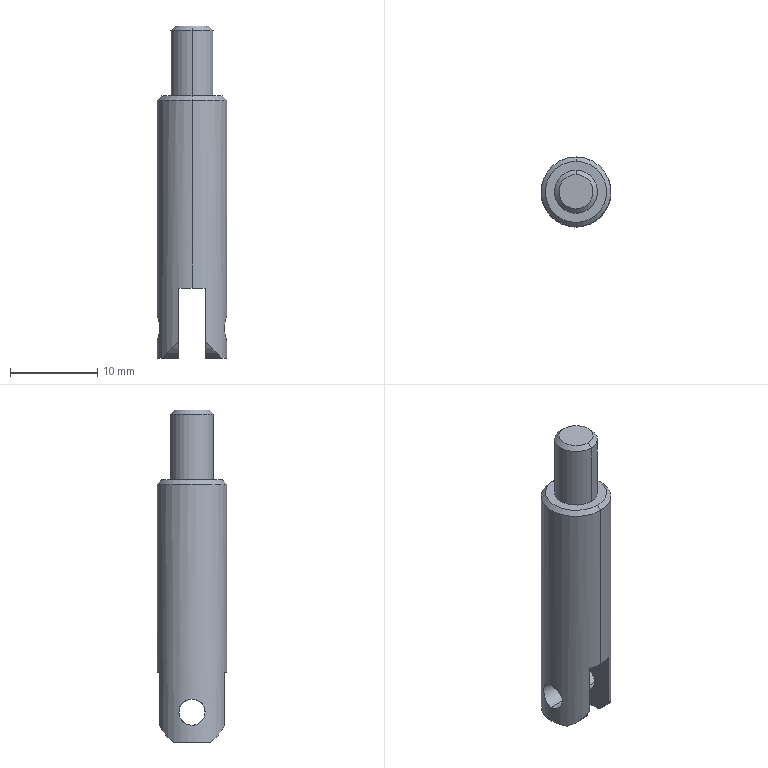Component | SolidWorks | GuideRod1-1 | 1 solid | 23 faces | box 8 x 8 x 38 mm | volume 1429 mm3 | cylinder 12 | plane 7 | cone 4 | commonest cylinder face diameters 8 x6 3 x4 4.917 x2
build123d program:
from build123d import *

# Parameters (mm, degrees)
SKETCH1_R           = 4
BOSS_EXTRUDE1_DEPTH = 30
SKETCH2_R           = 2.458
BOSS_EXTRUDE2_DEPTH = 8
CUT_EXTRUDE1_DEPTH  = 13
SKETCH5_W           = 16
SKETCH5_H           = 3
CUT_EXTRUDE2_DEPTH  = 13
SKETCH6_R           = 1.5
CUT_EXTRUDE3_DEPTH  = 13
CHAMFER1_SIZE       = 0.5


with BuildPart() as part:
    # Sketch1 → Boss-Extrude1 (new body)
    with BuildSketch(Plane.XY):
        Circle(SKETCH1_R)
    extrude(amount=BOSS_EXTRUDE1_DEPTH)

    # Sketch2 → Boss-Extrude2 (add)
    with BuildSketch(Plane(origin=(0, 0, 0), x_dir=(-1, 0, 0), z_dir=(0, 0, -1))):
        with Locations(Location((0, 0, 0), (0, 0, 180))):
            Circle(SKETCH2_R)
    extrude(amount=BOSS_EXTRUDE2_DEPTH)

    # Sketch4 → Cut-Extrude1 (cut, symmetric)
    with BuildSketch(Plane(origin=(0, 0, 0), x_dir=(1, 0, 0), z_dir=(0, 1, 0))):
        with BuildLine():
            Line((-4, -26.584), (-9.687, -26.584))
            Line((-9.687, -26.584), (-6.844, -32.06))
            Line((-6.844, -32.06), (5.728, -32.06))
            Line((5.728, -32.06), (7.666, -26.584))
            Line((7.666, -26.584), (4, -26.584))
            ThreePointArc((4, -26.584), (0, -30.584), (-4, -26.584))
        make_face()
    extrude(amount=CUT_EXTRUDE1_DEPTH, both=True, mode=Mode.SUBTRACT)

    # Sketch5 → Cut-Extrude2 (cut, symmetric)
    with BuildSketch(Plane(origin=(0, 0, 0), x_dir=(0, 0, -1), z_dir=(1, 0, 0))):
        with Locations((-30, 0)):
            Rectangle(SKETCH5_W, SKETCH5_H)
    extrude(amount=CUT_EXTRUDE2_DEPTH, both=True, mode=Mode.SUBTRACT)

    # Sketch6 → Cut-Extrude3 (cut, symmetric)
    with BuildSketch(Plane(origin=(0, 0, 0), x_dir=(1, 0, 0), z_dir=(0, 1, 0))):
        with Locations(Location((0, -26.584, 0), (0, 0, 270))):
            Circle(SKETCH6_R)
    extrude(amount=CUT_EXTRUDE3_DEPTH, both=True, mode=Mode.SUBTRACT)

    # Chamfer1
    chamfer1_edges = [part.edges().sort_by_distance(p)[0] for p in [
        (-4, 0, 0),
        (-2.458, 0, -8),
    ]]
    chamfer(chamfer1_edges, length=CHAMFER1_SIZE)


solid = part.part

# Placed as in the assembly
solid = solid.moved(Location((-15.928, -1.7, 62), (180, 0, -90)))
STEP:
#1=COLOUR_RGB('',0.7922,0.8196,0.9333);
#2=FILL_AREA_STYLE_COLOUR('',#1);
#3=FILL_AREA_STYLE('',(#2));
#4=SURFACE_STYLE_FILL_AREA(#3);
#5=SURFACE_SIDE_STYLE('',(#4));
#6=SURFACE_STYLE_USAGE(.BOTH.,#5);
#7=PRESENTATION_STYLE_ASSIGNMENT((#6));
#8=CARTESIAN_POINT('',(-0.6271,-0.144,2.756));
#9=VERTEX_POINT('',#8);
#10=CARTESIAN_POINT('',(-0.6271,0.01017,2.756));
#11=VERTEX_POINT('',#10);
#12=CARTESIAN_POINT('',(-0.6271,-0.06694,2.756));
#13=DIRECTION('',(0.,0.,1.));
#14=DIRECTION('',(0.,-1.,0.));
#15=AXIS2_PLACEMENT_3D('',#12,#13,#14);
#16=CIRCLE('',#15,0.07711);
#17=EDGE_CURVE('',#9,#11,#16,.T.);
#18=ORIENTED_EDGE('',*,*,#17,.F.);
#19=CARTESIAN_POINT('',(-0.6271,-0.1637,2.736));
#20=VERTEX_POINT('',#19);
#21=CARTESIAN_POINT('',(-0.6271,-0.144,2.756));
#22=DIRECTION('',(0.,-0.7071,-0.7071));
#23=VECTOR('',#22,39.37);
#24=LINE('',#21,#23);
#25=EDGE_CURVE('',#9,#20,#24,.T.);
#26=ORIENTED_EDGE('',*,*,#25,.T.);
#27=CARTESIAN_POINT('',(-0.6271,0.02985,2.736));
#28=VERTEX_POINT('',#27);
#29=CARTESIAN_POINT('',(-0.6271,-0.06694,2.736));
#30=DIRECTION('',(0.,0.,-1.));
#31=DIRECTION('',(0.,-1.,0.));
#32=AXIS2_PLACEMENT_3D('',#29,#30,#31);
#33=CIRCLE('',#32,0.09679);
#34=EDGE_CURVE('',#28,#20,#33,.T.);
#35=ORIENTED_EDGE('',*,*,#34,.F.);
#36=CARTESIAN_POINT('',(-0.6271,0.01017,2.756));
#37=DIRECTION('',(-0.,0.7071,-0.7071));
#38=VECTOR('',#37,39.37);
#39=LINE('',#36,#38);
#40=EDGE_CURVE('',#11,#28,#39,.T.);
#41=ORIENTED_EDGE('',*,*,#40,.F.);
#42=EDGE_LOOP('',(#18,#26,#35,#41));
#43=FACE_OUTER_BOUND('',#42,.T.);
#44=CARTESIAN_POINT('',(-0.6271,-0.06694,2.756));
#45=DIRECTION('',(0.,0.,-1.));
#46=DIRECTION('',(0.,1.,0.));
#47=AXIS2_PLACEMENT_3D('',#44,#45,#46);
#48=CONICAL_SURFACE('',#47,0.07711,0.7854);
#49=ADVANCED_FACE('',(#43),#48,.T.);
#50=CARTESIAN_POINT('',(-0.6271,-0.2047,2.441));
#51=VERTEX_POINT('',#50);
#52=CARTESIAN_POINT('',(-0.6271,0.07086,2.441));
#53=VERTEX_POINT('',#52);
#54=CARTESIAN_POINT('',(-0.6271,-0.06694,2.441));
#55=DIRECTION('',(0.,0.,1.));
#56=DIRECTION('',(0.,1.,0.));
#57=AXIS2_PLACEMENT_3D('',#54,#55,#56);
#58=CIRCLE('',#57,0.1378);
#59=EDGE_CURVE('',#51,#53,#58,.T.);
#60=ORIENTED_EDGE('',*,*,#59,.F.);
#61=CARTESIAN_POINT('',(-0.6271,-0.2244,2.421));
#62=VERTEX_POINT('',#61);
#63=CARTESIAN_POINT('',(-0.6271,-0.2244,2.421));
#64=DIRECTION('',(0.,-0.7071,-0.7071));
#65=VECTOR('',#64,39.37);
#66=LINE('',#63,#65);
#67=EDGE_CURVE('',#51,#62,#66,.T.);
#68=ORIENTED_EDGE('',*,*,#67,.T.);
#69=CARTESIAN_POINT('',(-0.6271,0.09054,2.421));
#70=VERTEX_POINT('',#69);
#71=CARTESIAN_POINT('',(-0.6271,-0.06694,2.421));
#72=DIRECTION('',(0.,0.,-1.));
#73=DIRECTION('',(0.,1.,0.));
#74=AXIS2_PLACEMENT_3D('',#71,#72,#73);
#75=CIRCLE('',#74,0.1575);
#76=EDGE_CURVE('',#70,#62,#75,.T.);
#77=ORIENTED_EDGE('',*,*,#76,.F.);
#78=CARTESIAN_POINT('',(-0.6271,0.09054,2.421));
#79=DIRECTION('',(-0.,0.7071,-0.7071));
#80=VECTOR('',#79,39.37);
#81=LINE('',#78,#80);
#82=EDGE_CURVE('',#53,#70,#81,.T.);
#83=ORIENTED_EDGE('',*,*,#82,.F.);
#84=EDGE_LOOP('',(#60,#68,#77,#83));
#85=FACE_OUTER_BOUND('',#84,.T.);
#86=CARTESIAN_POINT('',(-0.6271,-0.06694,2.421));
#87=DIRECTION('',(0.,0.,-1.));
#88=DIRECTION('',(0.,1.,0.));
#89=AXIS2_PLACEMENT_3D('',#86,#87,#88);
#90=CONICAL_SURFACE('',#89,0.1575,0.7854);
#91=ADVANCED_FACE('',(#85),#90,.T.);
#92=CARTESIAN_POINT('',(-0.7846,-0.06694,1.453));
#93=VERTEX_POINT('',#92);
#94=CARTESIAN_POINT('',(-0.7846,-0.06694,1.335));
#95=VERTEX_POINT('',#94);
#96=CARTESIAN_POINT('',(-0.7846,-0.06694,1.453));
#97=CARTESIAN_POINT('',(-0.7846,-0.0747,1.453));
#98=CARTESIAN_POINT('',(-0.784,-0.08253,1.452));
#99=CARTESIAN_POINT('',(-0.7824,-0.09323,1.447));
#100=CARTESIAN_POINT('',(-0.7818,-0.09668,1.445));
#101=CARTESIAN_POINT('',(-0.7804,-0.103,1.441));
#102=CARTESIAN_POINT('',(-0.7797,-0.106,1.439));
#103=CARTESIAN_POINT('',(-0.7774,-0.1142,1.431));
#104=CARTESIAN_POINT('',(-0.7759,-0.1185,1.424));
#105=CARTESIAN_POINT('',(-0.7743,-0.1229,1.413));
#106=CARTESIAN_POINT('',(-0.7738,-0.1241,1.41));
#107=CARTESIAN_POINT('',(-0.7732,-0.1256,1.402));
#108=CARTESIAN_POINT('',(-0.7731,-0.126,1.398));
#109=CARTESIAN_POINT('',(-0.7731,-0.126,1.387));
#110=CARTESIAN_POINT('',(-0.7737,-0.1244,1.379));
#111=CARTESIAN_POINT('',(-0.7759,-0.1185,1.364));
#112=CARTESIAN_POINT('',(-0.7774,-0.1141,1.358));
#113=CARTESIAN_POINT('',(-0.7797,-0.106,1.35));
#114=CARTESIAN_POINT('',(-0.7804,-0.103,1.347));
#115=CARTESIAN_POINT('',(-0.7818,-0.0966,1.343));
#116=CARTESIAN_POINT('',(-0.7824,-0.09323,1.341));
#117=CARTESIAN_POINT('',(-0.784,-0.08247,1.337));
#118=CARTESIAN_POINT('',(-0.7846,-0.07482,1.335));
#119=CARTESIAN_POINT('',(-0.7846,-0.06694,1.335));
#120=B_SPLINE_CURVE_WITH_KNOTS('',3,(#96,#97,#98,#99,#100,#101,#102,#103,#104,#105,#106,#107,#108,#109,#110,#111,#112,#113,#114,#115,#116,#117,#118,#119),.UNSPECIFIED.,.F.,.F.,(4,2,2,2,2,2,2,2,2,2,2,4),(0.004733,0.005325,0.005621,0.005916,0.006508,0.006804,0.0071,0.007691,0.008283,0.008578,0.008874,0.009466),.UNSPECIFIED.);
#121=EDGE_CURVE('',#93,#95,#120,.T.);
#122=ORIENTED_EDGE('',*,*,#121,.F.);
#123=CARTESIAN_POINT('',(-0.6861,-0.06694,1.453));
#124=VERTEX_POINT('',#123);
#125=CARTESIAN_POINT('',(-1.139,-0.06694,1.453));
#126=DIRECTION('',(1.,0.,0.));
#127=VECTOR('',#126,39.37);
#128=LINE('',#125,#127);
#129=EDGE_CURVE('',#93,#124,#128,.T.);
#130=ORIENTED_EDGE('',*,*,#129,.T.);
#131=CARTESIAN_POINT('',(-0.6861,-0.06694,1.335));
#132=VERTEX_POINT('',#131);
#133=CARTESIAN_POINT('',(-0.6861,-0.06694,1.394));
#134=DIRECTION('',(-1.,-0.,0.));
#135=DIRECTION('',(0.,0.,1.));
#136=AXIS2_PLACEMENT_3D('',#133,#134,#135);
#137=CIRCLE('',#136,0.05906);
#138=EDGE_CURVE('',#132,#124,#137,.T.);
#139=ORIENTED_EDGE('',*,*,#138,.F.);
#140=CARTESIAN_POINT('',(-1.139,-0.06694,1.335));
#141=DIRECTION('',(1.,0.,0.));
#142=VECTOR('',#141,39.37);
#143=LINE('',#140,#142);
#144=EDGE_CURVE('',#95,#132,#143,.T.);
#145=ORIENTED_EDGE('',*,*,#144,.F.);
#146=EDGE_LOOP('',(#122,#130,#139,#145));
#147=FACE_OUTER_BOUND('',#146,.T.);
#148=CARTESIAN_POINT('',(-1.139,-0.06694,1.394));
#149=DIRECTION('',(1.,0.,0.));
#150=DIRECTION('',(0.,0.,-1.));
#151=AXIS2_PLACEMENT_3D('',#148,#149,#150);
#152=CYLINDRICAL_SURFACE('',#151,0.05906);
#153=ADVANCED_FACE('',(#147),#152,.F.);
#154=CARTESIAN_POINT('',(-0.568,-0.06694,1.453));
#155=VERTEX_POINT('',#154);
#156=CARTESIAN_POINT('',(-0.568,-0.06694,1.335));
#157=VERTEX_POINT('',#156);
#158=CARTESIAN_POINT('',(-0.568,-0.06694,1.394));
#159=DIRECTION('',(1.,0.,0.));
#160=DIRECTION('',(0.,0.,-1.));
#161=AXIS2_PLACEMENT_3D('',#158,#159,#160);
#162=CIRCLE('',#161,0.05906);
#163=EDGE_CURVE('',#155,#157,#162,.T.);
#164=ORIENTED_EDGE('',*,*,#163,.F.);
#165=CARTESIAN_POINT('',(-0.4696,-0.06694,1.453));
#166=VERTEX_POINT('',#165);
#167=CARTESIAN_POINT('',(-1.139,-0.06694,1.453));
#168=DIRECTION('',(1.,0.,0.));
#169=VECTOR('',#168,39.37);
#170=LINE('',#167,#169);
#171=EDGE_CURVE('',#155,#166,#170,.T.);
#172=ORIENTED_EDGE('',*,*,#171,.T.);
#173=CARTESIAN_POINT('',(-0.4696,-0.06694,1.335));
#174=VERTEX_POINT('',#173);
#175=CARTESIAN_POINT('',(-0.4696,-0.06694,1.335));
#176=CARTESIAN_POINT('',(-0.4696,-0.07088,1.335));
#177=CARTESIAN_POINT('',(-0.4698,-0.07475,1.336));
#178=CARTESIAN_POINT('',(-0.4703,-0.08234,1.337));
#179=CARTESIAN_POINT('',(-0.4707,-0.08612,1.338));
#180=CARTESIAN_POINT('',(-0.4723,-0.09682,1.343));
#181=CARTESIAN_POINT('',(-0.4738,-0.1033,1.347));
#182=CARTESIAN_POINT('',(-0.4767,-0.1141,1.358));
#183=CARTESIAN_POINT('',(-0.4783,-0.1185,1.365));
#184=CARTESIAN_POINT('',(-0.4799,-0.1229,1.375));
#185=CARTESIAN_POINT('',(-0.4803,-0.1241,1.379));
#186=CARTESIAN_POINT('',(-0.4809,-0.1256,1.387));
#187=CARTESIAN_POINT('',(-0.4811,-0.126,1.39));
#188=CARTESIAN_POINT('',(-0.4811,-0.126,1.398));
#189=CARTESIAN_POINT('',(-0.4809,-0.1256,1.402));
#190=CARTESIAN_POINT('',(-0.4803,-0.1241,1.41));
#191=CARTESIAN_POINT('',(-0.4799,-0.1229,1.413));
#192=CARTESIAN_POINT('',(-0.4788,-0.1199,1.421));
#193=CARTESIAN_POINT('',(-0.4781,-0.1181,1.424));
#194=CARTESIAN_POINT('',(-0.4767,-0.1139,1.43));
#195=CARTESIAN_POINT('',(-0.476,-0.1114,1.433));
#196=CARTESIAN_POINT('',(-0.4745,-0.106,1.439));
#197=CARTESIAN_POINT('',(-0.4738,-0.103,1.441));
#198=CARTESIAN_POINT('',(-0.4724,-0.09664,1.446));
#199=CARTESIAN_POINT('',(-0.4718,-0.09319,1.447));
#200=CARTESIAN_POINT('',(-0.4702,-0.08254,1.452));
#201=CARTESIAN_POINT('',(-0.4696,-0.0747,1.453));
#202=CARTESIAN_POINT('',(-0.4696,-0.06694,1.453));
#203=B_SPLINE_CURVE_WITH_KNOTS('',3,(#175,#176,#177,#178,#179,#180,#181,#182,#183,#184,#185,#186,#187,#188,#189,#190,#191,#192,#193,#194,#195,#196,#197,#198,#199,#200,#201,#202),.UNSPECIFIED.,.F.,.F.,(4,2,2,2,2,2,2,2,2,2,2,2,2,4),(0.,0.0002958,0.0005917,0.001183,0.001775,0.002071,0.002367,0.002663,0.002958,0.003254,0.00355,0.003846,0.004142,0.004733),.UNSPECIFIED.);
#204=EDGE_CURVE('',#174,#166,#203,.T.);
#205=ORIENTED_EDGE('',*,*,#204,.F.);
#206=CARTESIAN_POINT('',(-1.139,-0.06694,1.335));
#207=DIRECTION('',(1.,0.,0.));
#208=VECTOR('',#207,39.37);
#209=LINE('',#206,#208);
#210=EDGE_CURVE('',#157,#174,#209,.T.);
#211=ORIENTED_EDGE('',*,*,#210,.F.);
#212=EDGE_LOOP('',(#164,#172,#205,#211));
#213=FACE_OUTER_BOUND('',#212,.T.);
#214=CARTESIAN_POINT('',(-1.139,-0.06694,1.394));
#215=DIRECTION('',(1.,0.,0.));
#216=DIRECTION('',(0.,0.,-1.));
#217=AXIS2_PLACEMENT_3D('',#214,#215,#216);
#218=CYLINDRICAL_SURFACE('',#217,0.05906);
#219=ADVANCED_FACE('',(#213),#218,.F.);
#220=ORIENTED_EDGE('',*,*,#34,.T.);
#221=CARTESIAN_POINT('',(-0.6271,-0.1637,2.441));
#222=VERTEX_POINT('',#221);
#223=CARTESIAN_POINT('',(-0.6271,-0.1637,2.756));
#224=DIRECTION('',(0.,0.,-1.));
#225=VECTOR('',#224,39.37);
#226=LINE('',#223,#225);
#227=EDGE_CURVE('',#20,#222,#226,.T.);
#228=ORIENTED_EDGE('',*,*,#227,.T.);
#229=CARTESIAN_POINT('',(-0.6271,0.02985,2.441));
#230=VERTEX_POINT('',#229);
#231=CARTESIAN_POINT('',(-0.6271,-0.06694,2.441));
#232=DIRECTION('',(0.,0.,1.));
#233=DIRECTION('',(0.,1.,0.));
#234=AXIS2_PLACEMENT_3D('',#231,#232,#233);
#235=CIRCLE('',#234,0.09679);
#236=EDGE_CURVE('',#222,#230,#235,.T.);
#237=ORIENTED_EDGE('',*,*,#236,.T.);
#238=CARTESIAN_POINT('',(-0.6271,0.02985,2.756));
#239=DIRECTION('',(0.,0.,-1.));
#240=VECTOR('',#239,39.37);
#241=LINE('',#238,#240);
#242=EDGE_CURVE('',#28,#230,#241,.T.);
#243=ORIENTED_EDGE('',*,*,#242,.F.);
#244=EDGE_LOOP('',(#220,#228,#237,#243));
#245=FACE_OUTER_BOUND('',#244,.T.);
#246=CARTESIAN_POINT('',(-0.6271,-0.06694,2.756));
#247=DIRECTION('',(0.,0.,-1.));
#248=DIRECTION('',(0.,1.,0.));
#249=AXIS2_PLACEMENT_3D('',#246,#247,#248);
#250=CYLINDRICAL_SURFACE('',#249,0.09679);
#251=ADVANCED_FACE('',(#245),#250,.T.);
#252=ORIENTED_EDGE('',*,*,#204,.T.);
#253=CARTESIAN_POINT('',(-0.4696,-0.06694,1.453));
#254=CARTESIAN_POINT('',(-0.4696,-0.05918,1.453));
#255=CARTESIAN_POINT('',(-0.4702,-0.05135,1.452));
#256=CARTESIAN_POINT('',(-0.4718,-0.04064,1.447));
#257=CARTESIAN_POINT('',(-0.4724,-0.03719,1.445));
#258=CARTESIAN_POINT('',(-0.4738,-0.03083,1.441));
#259=CARTESIAN_POINT('',(-0.4745,-0.02788,1.439));
#260=CARTESIAN_POINT('',(-0.4768,-0.01969,1.431));
#261=CARTESIAN_POINT('',(-0.4783,-0.01538,1.424));
#262=CARTESIAN_POINT('',(-0.4799,-0.01092,1.413));
#263=CARTESIAN_POINT('',(-0.4803,-0.009799,1.41));
#264=CARTESIAN_POINT('',(-0.4809,-0.008273,1.402));
#265=CARTESIAN_POINT('',(-0.4811,-0.00788,1.398));
#266=CARTESIAN_POINT('',(-0.4811,-0.007885,1.387));
#267=CARTESIAN_POINT('',(-0.4804,-0.009469,1.379));
#268=CARTESIAN_POINT('',(-0.4782,-0.0154,1.364));
#269=CARTESIAN_POINT('',(-0.4767,-0.01977,1.358));
#270=CARTESIAN_POINT('',(-0.4745,-0.0279,1.35));
#271=CARTESIAN_POINT('',(-0.4737,-0.03091,1.347));
#272=CARTESIAN_POINT('',(-0.4724,-0.03727,1.343));
#273=CARTESIAN_POINT('',(-0.4718,-0.04065,1.341));
#274=CARTESIAN_POINT('',(-0.4702,-0.05141,1.337));
#275=CARTESIAN_POINT('',(-0.4696,-0.05906,1.335));
#276=CARTESIAN_POINT('',(-0.4696,-0.06694,1.335));
#277=B_SPLINE_CURVE_WITH_KNOTS('',3,(#253,#254,#255,#256,#257,#258,#259,#260,#261,#262,#263,#264,#265,#266,#267,#268,#269,#270,#271,#272,#273,#274,#275,#276),.UNSPECIFIED.,.F.,.F.,(4,2,2,2,2,2,2,2,2,2,2,4),(0.004733,0.005325,0.005621,0.005916,0.006508,0.006804,0.0071,0.007691,0.008283,0.008578,0.008874,0.009466),.UNSPECIFIED.);
#278=EDGE_CURVE('',#166,#174,#277,.T.);
#279=ORIENTED_EDGE('',*,*,#278,.T.);
#280=EDGE_LOOP('',(#252,#279));
#281=FACE_BOUND('',#280,.T.);
#282=CARTESIAN_POINT('',(-0.568,0.07905,1.575));
#283=VERTEX_POINT('',#282);
#284=CARTESIAN_POINT('',(-0.6271,0.09054,1.575));
#285=VERTEX_POINT('',#284);
#286=CARTESIAN_POINT('',(-0.6271,-0.06694,1.575));
#287=DIRECTION('',(0.,0.,1.));
#288=DIRECTION('',(0.,-1.,0.));
#289=AXIS2_PLACEMENT_3D('',#286,#287,#288);
#290=CIRCLE('',#289,0.1575);
#291=EDGE_CURVE('',#283,#285,#290,.T.);
#292=ORIENTED_EDGE('',*,*,#291,.T.);
#293=CARTESIAN_POINT('',(-0.6271,0.09054,1.26));
#294=DIRECTION('',(0.,0.,1.));
#295=VECTOR('',#294,39.37);
#296=LINE('',#293,#295);
#297=EDGE_CURVE('',#285,#70,#296,.T.);
#298=ORIENTED_EDGE('',*,*,#297,.T.);
#299=ORIENTED_EDGE('',*,*,#76,.T.);
#300=CARTESIAN_POINT('',(-0.6271,-0.2244,1.575));
#301=VERTEX_POINT('',#300);
#302=CARTESIAN_POINT('',(-0.6271,-0.2244,1.26));
#303=DIRECTION('',(0.,0.,1.));
#304=VECTOR('',#303,39.37);
#305=LINE('',#302,#304);
#306=EDGE_CURVE('',#301,#62,#305,.T.);
#307=ORIENTED_EDGE('',*,*,#306,.F.);
#308=CARTESIAN_POINT('',(-0.568,-0.2129,1.575));
#309=VERTEX_POINT('',#308);
#310=CARTESIAN_POINT('',(-0.6271,-0.06694,1.575));
#311=DIRECTION('',(0.,0.,1.));
#312=DIRECTION('',(0.,-1.,0.));
#313=AXIS2_PLACEMENT_3D('',#310,#311,#312);
#314=CIRCLE('',#313,0.1575);
#315=EDGE_CURVE('',#301,#309,#314,.T.);
#316=ORIENTED_EDGE('',*,*,#315,.T.);
#317=CARTESIAN_POINT('',(-0.568,-0.2129,1.335));
#318=VERTEX_POINT('',#317);
#319=CARTESIAN_POINT('',(-0.568,-0.2129,1.26));
#320=DIRECTION('',(0.,0.,-1.));
#321=VECTOR('',#320,39.37);
#322=LINE('',#319,#321);
#323=EDGE_CURVE('',#309,#318,#322,.T.);
#324=ORIENTED_EDGE('',*,*,#323,.T.);
#325=CARTESIAN_POINT('',(-0.4926,-0.1489,1.26));
#326=VERTEX_POINT('',#325);
#327=CARTESIAN_POINT('',(-0.568,-0.2129,1.335));
#328=CARTESIAN_POINT('',(-0.5364,-0.2001,1.304));
#329=CARTESIAN_POINT('',(-0.5104,-0.178,1.278));
#330=CARTESIAN_POINT('',(-0.4926,-0.1489,1.26));
#331=(BOUNDED_CURVE()B_SPLINE_CURVE(3,(#327,#328,#329,#330),.UNSPECIFIED.,.F.,.T.)B_SPLINE_CURVE_WITH_KNOTS((4,4),(1.955,2.594),.UNSPECIFIED.)CURVE()GEOMETRIC_REPRESENTATION_ITEM()RATIONAL_B_SPLINE_CURVE((1.,0.9662,0.9662,1.))REPRESENTATION_ITEM(''));
#332=EDGE_CURVE('',#318,#326,#331,.T.);
#333=ORIENTED_EDGE('',*,*,#332,.T.);
#334=CARTESIAN_POINT('',(-0.4926,0.015,1.26));
#335=VERTEX_POINT('',#334);
#336=CARTESIAN_POINT('',(-0.6271,-0.06694,1.26));
#337=DIRECTION('',(0.,0.,-1.));
#338=DIRECTION('',(0.,1.,0.));
#339=AXIS2_PLACEMENT_3D('',#336,#337,#338);
#340=CIRCLE('',#339,0.1575);
#341=EDGE_CURVE('',#335,#326,#340,.T.);
#342=ORIENTED_EDGE('',*,*,#341,.F.);
#343=CARTESIAN_POINT('',(-0.568,0.07905,1.335));
#344=VERTEX_POINT('',#343);
#345=CARTESIAN_POINT('',(-0.4926,0.015,1.26));
#346=CARTESIAN_POINT('',(-0.5104,0.04416,1.278));
#347=CARTESIAN_POINT('',(-0.5364,0.06625,1.304));
#348=CARTESIAN_POINT('',(-0.568,0.07905,1.335));
#349=(BOUNDED_CURVE()B_SPLINE_CURVE(3,(#345,#346,#347,#348),.UNSPECIFIED.,.F.,.F.)B_SPLINE_CURVE_WITH_KNOTS((4,4),(3.689,4.328),.UNSPECIFIED.)CURVE()GEOMETRIC_REPRESENTATION_ITEM()RATIONAL_B_SPLINE_CURVE((1.,0.9662,0.9662,1.))REPRESENTATION_ITEM(''));
#350=EDGE_CURVE('',#335,#344,#349,.T.);
#351=ORIENTED_EDGE('',*,*,#350,.T.);
#352=CARTESIAN_POINT('',(-0.568,0.07905,1.26));
#353=DIRECTION('',(0.,0.,1.));
#354=VECTOR('',#353,39.37);
#355=LINE('',#352,#354);
#356=EDGE_CURVE('',#344,#283,#355,.T.);
#357=ORIENTED_EDGE('',*,*,#356,.T.);
#358=EDGE_LOOP('',(#292,#298,#299,#307,#316,#324,#333,#342,#351,#357));
#359=FACE_OUTER_BOUND('',#358,.T.);
#360=CARTESIAN_POINT('',(-0.6271,-0.06694,1.26));
#361=DIRECTION('',(0.,0.,1.));
#362=DIRECTION('',(0.,-1.,0.));
#363=AXIS2_PLACEMENT_3D('',#360,#361,#362);
#364=CYLINDRICAL_SURFACE('',#363,0.1575);
#365=ADVANCED_FACE('',(#281,#359),#364,.T.);
#366=CARTESIAN_POINT('',(-0.6861,-0.1489,1.26));
#367=VERTEX_POINT('',#366);
#368=CARTESIAN_POINT('',(-0.6861,0.015,1.26));
#369=VERTEX_POINT('',#368);
#370=CARTESIAN_POINT('',(-0.6861,-0.06694,1.26));
#371=DIRECTION('',(-0.,1.,0.));
#372=VECTOR('',#371,39.37);
#373=LINE('',#370,#372);
#374=EDGE_CURVE('',#367,#369,#373,.T.);
#375=ORIENTED_EDGE('',*,*,#374,.F.);
#376=CARTESIAN_POINT('',(-0.7616,-0.1489,1.26));
#377=VERTEX_POINT('',#376);
#378=CARTESIAN_POINT('',(-1.139,-0.1489,1.26));
#379=DIRECTION('',(1.,0.,0.));
#380=VECTOR('',#379,39.37);
#381=LINE('',#378,#380);
#382=EDGE_CURVE('',#377,#367,#381,.T.);
#383=ORIENTED_EDGE('',*,*,#382,.F.);
#384=CARTESIAN_POINT('',(-0.7616,0.015,1.26));
#385=VERTEX_POINT('',#384);
#386=CARTESIAN_POINT('',(-0.6271,-0.06694,1.26));
#387=DIRECTION('',(0.,0.,-1.));
#388=DIRECTION('',(0.,1.,0.));
#389=AXIS2_PLACEMENT_3D('',#386,#387,#388);
#390=CIRCLE('',#389,0.1575);
#391=EDGE_CURVE('',#377,#385,#390,.T.);
#392=ORIENTED_EDGE('',*,*,#391,.T.);
#393=CARTESIAN_POINT('',(-1.139,0.015,1.26));
#394=DIRECTION('',(-1.,-0.,0.));
#395=VECTOR('',#394,39.37);
#396=LINE('',#393,#395);
#397=EDGE_CURVE('',#369,#385,#396,.T.);
#398=ORIENTED_EDGE('',*,*,#397,.F.);
#399=EDGE_LOOP('',(#375,#383,#392,#398));
#400=FACE_OUTER_BOUND('',#399,.T.);
#401=CARTESIAN_POINT('',(-0.6271,-0.06694,1.26));
#402=DIRECTION('',(0.,0.,-1.));
#403=DIRECTION('',(-0.,1.,0.));
#404=AXIS2_PLACEMENT_3D('',#401,#402,#403);
#405=PLANE('',#404);
#406=ADVANCED_FACE('',(#400),#405,.T.);
#407=ORIENTED_EDGE('',*,*,#382,.T.);
#408=CARTESIAN_POINT('',(-0.6861,-0.2129,1.335));
#409=VERTEX_POINT('',#408);
#410=CARTESIAN_POINT('',(-0.6861,-0.06694,1.394));
#411=DIRECTION('',(-1.,-0.,0.));
#412=DIRECTION('',(0.,0.,1.));
#413=AXIS2_PLACEMENT_3D('',#410,#411,#412);
#414=CIRCLE('',#413,0.1575);
#415=EDGE_CURVE('',#367,#409,#414,.T.);
#416=ORIENTED_EDGE('',*,*,#415,.T.);
#417=CARTESIAN_POINT('',(-0.7616,-0.1489,1.26));
#418=CARTESIAN_POINT('',(-0.7438,-0.178,1.278));
#419=CARTESIAN_POINT('',(-0.7178,-0.2001,1.304));
#420=CARTESIAN_POINT('',(-0.6861,-0.2129,1.335));
#421=(BOUNDED_CURVE()B_SPLINE_CURVE(3,(#417,#418,#419,#420),.UNSPECIFIED.,.F.,.T.)B_SPLINE_CURVE_WITH_KNOTS((4,4),(3.689,4.328),.UNSPECIFIED.)CURVE()GEOMETRIC_REPRESENTATION_ITEM()RATIONAL_B_SPLINE_CURVE((1.,0.9662,0.9662,1.))REPRESENTATION_ITEM(''));
#422=EDGE_CURVE('',#377,#409,#421,.T.);
#423=ORIENTED_EDGE('',*,*,#422,.F.);
#424=EDGE_LOOP('',(#407,#416,#423));
#425=FACE_OUTER_BOUND('',#424,.T.);
#426=CARTESIAN_POINT('',(-1.139,-0.06694,1.394));
#427=DIRECTION('',(1.,0.,0.));
#428=DIRECTION('',(0.,0.,-1.));
#429=AXIS2_PLACEMENT_3D('',#426,#427,#428);
#430=CYLINDRICAL_SURFACE('',#429,0.1575);
#431=ADVANCED_FACE('',(#425),#430,.T.);
#432=CARTESIAN_POINT('',(-0.6861,0.07905,1.335));
#433=VERTEX_POINT('',#432);
#434=CARTESIAN_POINT('',(-0.6861,0.07905,1.335));
#435=CARTESIAN_POINT('',(-0.7178,0.06625,1.304));
#436=CARTESIAN_POINT('',(-0.7438,0.04416,1.278));
#437=CARTESIAN_POINT('',(-0.7616,0.015,1.26));
#438=(BOUNDED_CURVE()B_SPLINE_CURVE(3,(#434,#435,#436,#437),.UNSPECIFIED.,.F.,.F.)B_SPLINE_CURVE_WITH_KNOTS((4,4),(1.955,2.594),.UNSPECIFIED.)CURVE()GEOMETRIC_REPRESENTATION_ITEM()RATIONAL_B_SPLINE_CURVE((1.,0.9662,0.9662,1.))REPRESENTATION_ITEM(''));
#439=EDGE_CURVE('',#433,#385,#438,.T.);
#440=ORIENTED_EDGE('',*,*,#439,.F.);
#441=CARTESIAN_POINT('',(-0.6861,-0.06694,1.394));
#442=DIRECTION('',(-1.,-0.,0.));
#443=DIRECTION('',(0.,0.,1.));
#444=AXIS2_PLACEMENT_3D('',#441,#442,#443);
#445=CIRCLE('',#444,0.1575);
#446=EDGE_CURVE('',#433,#369,#445,.T.);
#447=ORIENTED_EDGE('',*,*,#446,.T.);
#448=ORIENTED_EDGE('',*,*,#397,.T.);
#449=EDGE_LOOP('',(#440,#447,#448));
#450=FACE_OUTER_BOUND('',#449,.T.);
#451=CARTESIAN_POINT('',(-1.139,-0.06694,1.394));
#452=DIRECTION('',(1.,0.,0.));
#453=DIRECTION('',(0.,0.,-1.));
#454=AXIS2_PLACEMENT_3D('',#451,#452,#453);
#455=CYLINDRICAL_SURFACE('',#454,0.1575);
#456=ADVANCED_FACE('',(#450),#455,.T.);
#457=CARTESIAN_POINT('',(-0.6271,-0.06694,2.441));
#458=DIRECTION('',(0.,0.,1.));
#459=DIRECTION('',(0.,1.,0.));
#460=AXIS2_PLACEMENT_3D('',#457,#458,#459);
#461=CIRCLE('',#460,0.1378);
#462=EDGE_CURVE('',#53,#51,#461,.T.);
#463=ORIENTED_EDGE('',*,*,#462,.T.);
#464=ORIENTED_EDGE('',*,*,#59,.T.);
#465=EDGE_LOOP('',(#463,#464));
#466=FACE_OUTER_BOUND('',#465,.T.);
#467=CARTESIAN_POINT('',(-0.6271,-0.06694,2.441));
#468=DIRECTION('',(0.,0.,1.));
#469=DIRECTION('',(0.,1.,0.));
#470=AXIS2_PLACEMENT_3D('',#467,#468,#469);
#471=CIRCLE('',#470,0.09679);
#472=EDGE_CURVE('',#230,#222,#471,.T.);
#473=ORIENTED_EDGE('',*,*,#472,.F.);
#474=ORIENTED_EDGE('',*,*,#236,.F.);
#475=EDGE_LOOP('',(#473,#474));
#476=FACE_BOUND('',#475,.T.);
#477=CARTESIAN_POINT('',(-0.6271,-0.06694,2.441));
#478=DIRECTION('',(0.,0.,-1.));
#479=DIRECTION('',(-0.,1.,0.));
#480=AXIS2_PLACEMENT_3D('',#477,#478,#479);
#481=PLANE('',#480);
#482=ADVANCED_FACE('',(#466,#476),#481,.F.);
#483=ORIENTED_EDGE('',*,*,#297,.F.);
#484=CARTESIAN_POINT('',(-0.6861,0.07905,1.575));
#485=VERTEX_POINT('',#484);
#486=CARTESIAN_POINT('',(-0.6271,-0.06694,1.575));
#487=DIRECTION('',(0.,0.,1.));
#488=DIRECTION('',(0.,-1.,0.));
#489=AXIS2_PLACEMENT_3D('',#486,#487,#488);
#490=CIRCLE('',#489,0.1575);
#491=EDGE_CURVE('',#285,#485,#490,.T.);
#492=ORIENTED_EDGE('',*,*,#491,.T.);
#493=CARTESIAN_POINT('',(-0.6861,0.07905,1.26));
#494=DIRECTION('',(0.,0.,-1.));
#495=VECTOR('',#494,39.37);
#496=LINE('',#493,#495);
#497=EDGE_CURVE('',#485,#433,#496,.T.);
#498=ORIENTED_EDGE('',*,*,#497,.T.);
#499=ORIENTED_EDGE('',*,*,#439,.T.);
#500=ORIENTED_EDGE('',*,*,#391,.F.);
#501=ORIENTED_EDGE('',*,*,#422,.T.);
#502=CARTESIAN_POINT('',(-0.6861,-0.2129,1.575));
#503=VERTEX_POINT('',#502);
#504=CARTESIAN_POINT('',(-0.6861,-0.2129,1.26));
#505=DIRECTION('',(0.,0.,1.));
#506=VECTOR('',#505,39.37);
#507=LINE('',#504,#506);
#508=EDGE_CURVE('',#409,#503,#507,.T.);
#509=ORIENTED_EDGE('',*,*,#508,.T.);
#510=CARTESIAN_POINT('',(-0.6271,-0.06694,1.575));
#511=DIRECTION('',(0.,0.,1.));
#512=DIRECTION('',(0.,-1.,0.));
#513=AXIS2_PLACEMENT_3D('',#510,#511,#512);
#514=CIRCLE('',#513,0.1575);
#515=EDGE_CURVE('',#503,#301,#514,.T.);
#516=ORIENTED_EDGE('',*,*,#515,.T.);
#517=ORIENTED_EDGE('',*,*,#306,.T.);
#518=CARTESIAN_POINT('',(-0.6271,-0.06694,2.421));
#519=DIRECTION('',(0.,0.,-1.));
#520=DIRECTION('',(0.,1.,0.));
#521=AXIS2_PLACEMENT_3D('',#518,#519,#520);
#522=CIRCLE('',#521,0.1575);
#523=EDGE_CURVE('',#62,#70,#522,.T.);
#524=ORIENTED_EDGE('',*,*,#523,.T.);
#525=EDGE_LOOP('',(#483,#492,#498,#499,#500,#501,#509,#516,#517,#524));
#526=FACE_OUTER_BOUND('',#525,.T.);
#527=CARTESIAN_POINT('',(-0.7846,-0.06694,1.335));
#528=CARTESIAN_POINT('',(-0.7846,-0.063,1.335));
#529=CARTESIAN_POINT('',(-0.7844,-0.05913,1.336));
#530=CARTESIAN_POINT('',(-0.7839,-0.05153,1.337));
#531=CARTESIAN_POINT('',(-0.7834,-0.04776,1.338));
#532=CARTESIAN_POINT('',(-0.7819,-0.03705,1.343));
#533=CARTESIAN_POINT('',(-0.7804,-0.03055,1.347));
#534=CARTESIAN_POINT('',(-0.7774,-0.01976,1.358));
#535=CARTESIAN_POINT('',(-0.7759,-0.01538,1.365));
#536=CARTESIAN_POINT('',(-0.7743,-0.01095,1.375));
#537=CARTESIAN_POINT('',(-0.7738,-0.009798,1.379));
#538=CARTESIAN_POINT('',(-0.7732,-0.008267,1.387));
#539=CARTESIAN_POINT('',(-0.7731,-0.007883,1.39));
#540=CARTESIAN_POINT('',(-0.7731,-0.007879,1.398));
#541=CARTESIAN_POINT('',(-0.7732,-0.008272,1.402));
#542=CARTESIAN_POINT('',(-0.7738,-0.009798,1.41));
#543=CARTESIAN_POINT('',(-0.7743,-0.01093,1.413));
#544=CARTESIAN_POINT('',(-0.7754,-0.01393,1.421));
#545=CARTESIAN_POINT('',(-0.776,-0.01575,1.424));
#546=CARTESIAN_POINT('',(-0.7774,-0.02001,1.43));
#547=CARTESIAN_POINT('',(-0.7782,-0.02249,1.433));
#548=CARTESIAN_POINT('',(-0.7797,-0.0279,1.439));
#549=CARTESIAN_POINT('',(-0.7804,-0.03085,1.441));
#550=CARTESIAN_POINT('',(-0.7818,-0.03723,1.446));
#551=CARTESIAN_POINT('',(-0.7824,-0.04068,1.447));
#552=CARTESIAN_POINT('',(-0.784,-0.05134,1.452));
#553=CARTESIAN_POINT('',(-0.7846,-0.05917,1.453));
#554=CARTESIAN_POINT('',(-0.7846,-0.06694,1.453));
#555=B_SPLINE_CURVE_WITH_KNOTS('',3,(#527,#528,#529,#530,#531,#532,#533,#534,#535,#536,#537,#538,#539,#540,#541,#542,#543,#544,#545,#546,#547,#548,#549,#550,#551,#552,#553,#554),.UNSPECIFIED.,.F.,.F.,(4,2,2,2,2,2,2,2,2,2,2,2,2,4),(0.,0.0002958,0.0005917,0.001183,0.001775,0.002071,0.002367,0.002663,0.002958,0.003254,0.00355,0.003846,0.004142,0.004733),.UNSPECIFIED.);
#556=EDGE_CURVE('',#95,#93,#555,.T.);
#557=ORIENTED_EDGE('',*,*,#556,.T.);
#558=ORIENTED_EDGE('',*,*,#121,.T.);
#559=EDGE_LOOP('',(#557,#558));
#560=FACE_BOUND('',#559,.T.);
#561=CARTESIAN_POINT('',(-0.6271,-0.06694,1.26));
#562=DIRECTION('',(0.,0.,1.));
#563=DIRECTION('',(0.,-1.,0.));
#564=AXIS2_PLACEMENT_3D('',#561,#562,#563);
#565=CYLINDRICAL_SURFACE('',#564,0.1575);
#566=ADVANCED_FACE('',(#526,#560),#565,.T.);
#567=CARTESIAN_POINT('',(-0.568,0.015,1.26));
#568=VERTEX_POINT('',#567);
#569=CARTESIAN_POINT('',(-0.568,-0.1489,1.26));
#570=VERTEX_POINT('',#569);
#571=CARTESIAN_POINT('',(-0.568,-0.06694,1.26));
#572=DIRECTION('',(0.,-1.,0.));
#573=VECTOR('',#572,39.37);
#574=LINE('',#571,#573);
#575=EDGE_CURVE('',#568,#570,#574,.T.);
#576=ORIENTED_EDGE('',*,*,#575,.F.);
#577=CARTESIAN_POINT('',(-1.139,0.015,1.26));
#578=DIRECTION('',(-1.,-0.,0.));
#579=VECTOR('',#578,39.37);
#580=LINE('',#577,#579);
#581=EDGE_CURVE('',#335,#568,#580,.T.);
#582=ORIENTED_EDGE('',*,*,#581,.F.);
#583=ORIENTED_EDGE('',*,*,#341,.T.);
#584=CARTESIAN_POINT('',(-1.139,-0.1489,1.26));
#585=DIRECTION('',(1.,0.,0.));
#586=VECTOR('',#585,39.37);
#587=LINE('',#584,#586);
#588=EDGE_CURVE('',#570,#326,#587,.T.);
#589=ORIENTED_EDGE('',*,*,#588,.F.);
#590=EDGE_LOOP('',(#576,#582,#583,#589));
#591=FACE_OUTER_BOUND('',#590,.T.);
#592=CARTESIAN_POINT('',(-0.6271,-0.06694,1.26));
#593=DIRECTION('',(0.,0.,-1.));
#594=DIRECTION('',(-0.,1.,0.));
#595=AXIS2_PLACEMENT_3D('',#592,#593,#594);
#596=PLANE('',#595);
#597=ADVANCED_FACE('',(#591),#596,.T.);
#598=ORIENTED_EDGE('',*,*,#227,.F.);
#599=CARTESIAN_POINT('',(-0.6271,-0.06694,2.736));
#600=DIRECTION('',(0.,0.,-1.));
#601=DIRECTION('',(0.,-1.,0.));
#602=AXIS2_PLACEMENT_3D('',#599,#600,#601);
#603=CIRCLE('',#602,0.09679);
#604=EDGE_CURVE('',#20,#28,#603,.T.);
#605=ORIENTED_EDGE('',*,*,#604,.T.);
#606=ORIENTED_EDGE('',*,*,#242,.T.);
#607=ORIENTED_EDGE('',*,*,#472,.T.);
#608=EDGE_LOOP('',(#598,#605,#606,#607));
#609=FACE_OUTER_BOUND('',#608,.T.);
#610=CARTESIAN_POINT('',(-0.6271,-0.06694,2.756));
#611=DIRECTION('',(0.,0.,-1.));
#612=DIRECTION('',(0.,1.,0.));
#613=AXIS2_PLACEMENT_3D('',#610,#611,#612);
#614=CYLINDRICAL_SURFACE('',#613,0.09679);
#615=ADVANCED_FACE('',(#609),#614,.T.);
#616=CARTESIAN_POINT('',(-0.6271,-0.06694,2.756));
#617=DIRECTION('',(0.,0.,1.));
#618=DIRECTION('',(0.,-1.,0.));
#619=AXIS2_PLACEMENT_3D('',#616,#617,#618);
#620=CIRCLE('',#619,0.07711);
#621=EDGE_CURVE('',#11,#9,#620,.T.);
#622=ORIENTED_EDGE('',*,*,#621,.T.);
#623=ORIENTED_EDGE('',*,*,#17,.T.);
#624=EDGE_LOOP('',(#622,#623));
#625=FACE_OUTER_BOUND('',#624,.T.);
#626=CARTESIAN_POINT('',(-0.6271,-0.06694,2.756));
#627=DIRECTION('',(0.,0.,1.));
#628=DIRECTION('',(0.,-1.,0.));
#629=AXIS2_PLACEMENT_3D('',#626,#627,#628);
#630=PLANE('',#629);
#631=ADVANCED_FACE('',(#625),#630,.T.);
#632=ORIENTED_EDGE('',*,*,#332,.F.);
#633=CARTESIAN_POINT('',(-0.568,-0.06694,1.394));
#634=DIRECTION('',(1.,0.,0.));
#635=DIRECTION('',(0.,0.,-1.));
#636=AXIS2_PLACEMENT_3D('',#633,#634,#635);
#637=CIRCLE('',#636,0.1575);
#638=EDGE_CURVE('',#318,#570,#637,.T.);
#639=ORIENTED_EDGE('',*,*,#638,.T.);
#640=ORIENTED_EDGE('',*,*,#588,.T.);
#641=EDGE_LOOP('',(#632,#639,#640));
#642=FACE_OUTER_BOUND('',#641,.T.);
#643=CARTESIAN_POINT('',(-1.139,-0.06694,1.394));
#644=DIRECTION('',(1.,0.,0.));
#645=DIRECTION('',(0.,0.,-1.));
#646=AXIS2_PLACEMENT_3D('',#643,#644,#645);
#647=CYLINDRICAL_SURFACE('',#646,0.1575);
#648=ADVANCED_FACE('',(#642),#647,.T.);
#649=ORIENTED_EDGE('',*,*,#581,.T.);
#650=CARTESIAN_POINT('',(-0.568,-0.06694,1.394));
#651=DIRECTION('',(1.,0.,0.));
#652=DIRECTION('',(0.,0.,-1.));
#653=AXIS2_PLACEMENT_3D('',#650,#651,#652);
#654=CIRCLE('',#653,0.1575);
#655=EDGE_CURVE('',#568,#344,#654,.T.);
#656=ORIENTED_EDGE('',*,*,#655,.T.);
#657=ORIENTED_EDGE('',*,*,#350,.F.);
#658=EDGE_LOOP('',(#649,#656,#657));
#659=FACE_OUTER_BOUND('',#658,.T.);
#660=CARTESIAN_POINT('',(-1.139,-0.06694,1.394));
#661=DIRECTION('',(1.,0.,0.));
#662=DIRECTION('',(0.,0.,-1.));
#663=AXIS2_PLACEMENT_3D('',#660,#661,#662);
#664=CYLINDRICAL_SURFACE('',#663,0.1575);
#665=ADVANCED_FACE('',(#659),#664,.T.);
#666=CARTESIAN_POINT('',(-0.568,-0.5787,1.575));
#667=DIRECTION('',(-0.,1.,0.));
#668=VECTOR('',#667,39.37);
#669=LINE('',#666,#668);
#670=EDGE_CURVE('',#309,#283,#669,.T.);
#671=ORIENTED_EDGE('',*,*,#670,.F.);
#672=ORIENTED_EDGE('',*,*,#315,.F.);
#673=ORIENTED_EDGE('',*,*,#515,.F.);
#674=CARTESIAN_POINT('',(-0.6861,-0.5787,1.575));
#675=DIRECTION('',(-0.,1.,0.));
#676=VECTOR('',#675,39.37);
#677=LINE('',#674,#676);
#678=EDGE_CURVE('',#503,#485,#677,.T.);
#679=ORIENTED_EDGE('',*,*,#678,.T.);
#680=ORIENTED_EDGE('',*,*,#491,.F.);
#681=ORIENTED_EDGE('',*,*,#291,.F.);
#682=EDGE_LOOP('',(#671,#672,#673,#679,#680,#681));
#683=FACE_OUTER_BOUND('',#682,.T.);
#684=CARTESIAN_POINT('',(-0.568,-0.5787,1.575));
#685=DIRECTION('',(0.,0.,1.));
#686=DIRECTION('',(0.,-1.,0.));
#687=AXIS2_PLACEMENT_3D('',#684,#685,#686);
#688=PLANE('',#687);
#689=ADVANCED_FACE('',(#683),#688,.F.);
#690=ORIENTED_EDGE('',*,*,#138,.T.);
#691=CARTESIAN_POINT('',(-0.6861,-0.06694,1.394));
#692=DIRECTION('',(-1.,-0.,0.));
#693=DIRECTION('',(0.,0.,1.));
#694=AXIS2_PLACEMENT_3D('',#691,#692,#693);
#695=CIRCLE('',#694,0.05906);
#696=EDGE_CURVE('',#124,#132,#695,.T.);
#697=ORIENTED_EDGE('',*,*,#696,.T.);
#698=EDGE_LOOP('',(#690,#697));
#699=FACE_BOUND('',#698,.T.);
#700=ORIENTED_EDGE('',*,*,#415,.F.);
#701=ORIENTED_EDGE('',*,*,#374,.T.);
#702=ORIENTED_EDGE('',*,*,#446,.F.);
#703=ORIENTED_EDGE('',*,*,#497,.F.);
#704=ORIENTED_EDGE('',*,*,#678,.F.);
#705=ORIENTED_EDGE('',*,*,#508,.F.);
#706=EDGE_LOOP('',(#700,#701,#702,#703,#704,#705));
#707=FACE_OUTER_BOUND('',#706,.T.);
#708=CARTESIAN_POINT('',(-0.6861,-0.5787,0.9449));
#709=DIRECTION('',(-1.,-0.,0.));
#710=DIRECTION('',(0.,0.,1.));
#711=AXIS2_PLACEMENT_3D('',#708,#709,#710);
#712=PLANE('',#711);
#713=ADVANCED_FACE('',(#699,#707),#712,.F.);
#714=CARTESIAN_POINT('',(-0.568,-0.06694,1.394));
#715=DIRECTION('',(1.,0.,0.));
#716=DIRECTION('',(0.,0.,-1.));
#717=AXIS2_PLACEMENT_3D('',#714,#715,#716);
#718=CIRCLE('',#717,0.05906);
#719=EDGE_CURVE('',#157,#155,#718,.T.);
#720=ORIENTED_EDGE('',*,*,#719,.T.);
#721=ORIENTED_EDGE('',*,*,#163,.T.);
#722=EDGE_LOOP('',(#720,#721));
#723=FACE_BOUND('',#722,.T.);
#724=ORIENTED_EDGE('',*,*,#670,.T.);
#725=ORIENTED_EDGE('',*,*,#356,.F.);
#726=ORIENTED_EDGE('',*,*,#655,.F.);
#727=ORIENTED_EDGE('',*,*,#575,.T.);
#728=ORIENTED_EDGE('',*,*,#638,.F.);
#729=ORIENTED_EDGE('',*,*,#323,.F.);
#730=EDGE_LOOP('',(#724,#725,#726,#727,#728,#729));
#731=FACE_OUTER_BOUND('',#730,.T.);
#732=CARTESIAN_POINT('',(-0.568,-0.5787,0.9449));
#733=DIRECTION('',(1.,0.,0.));
#734=DIRECTION('',(0.,0.,-1.));
#735=AXIS2_PLACEMENT_3D('',#732,#733,#734);
#736=PLANE('',#735);
#737=ADVANCED_FACE('',(#723,#731),#736,.F.);
#738=ORIENTED_EDGE('',*,*,#171,.F.);
#739=ORIENTED_EDGE('',*,*,#719,.F.);
#740=ORIENTED_EDGE('',*,*,#210,.T.);
#741=ORIENTED_EDGE('',*,*,#278,.F.);
#742=EDGE_LOOP('',(#738,#739,#740,#741));
#743=FACE_OUTER_BOUND('',#742,.T.);
#744=CARTESIAN_POINT('',(-1.139,-0.06694,1.394));
#745=DIRECTION('',(1.,0.,0.));
#746=DIRECTION('',(0.,0.,-1.));
#747=AXIS2_PLACEMENT_3D('',#744,#745,#746);
#748=CYLINDRICAL_SURFACE('',#747,0.05906);
#749=ADVANCED_FACE('',(#743),#748,.F.);
#750=ORIENTED_EDGE('',*,*,#129,.F.);
#751=ORIENTED_EDGE('',*,*,#556,.F.);
#752=ORIENTED_EDGE('',*,*,#144,.T.);
#753=ORIENTED_EDGE('',*,*,#696,.F.);
#754=EDGE_LOOP('',(#750,#751,#752,#753));
#755=FACE_OUTER_BOUND('',#754,.T.);
#756=CARTESIAN_POINT('',(-1.139,-0.06694,1.394));
#757=DIRECTION('',(1.,0.,0.));
#758=DIRECTION('',(0.,0.,-1.));
#759=AXIS2_PLACEMENT_3D('',#756,#757,#758);
#760=CYLINDRICAL_SURFACE('',#759,0.05906);
#761=ADVANCED_FACE('',(#755),#760,.F.);
#762=ORIENTED_EDGE('',*,*,#67,.F.);
#763=ORIENTED_EDGE('',*,*,#462,.F.);
#764=ORIENTED_EDGE('',*,*,#82,.T.);
#765=ORIENTED_EDGE('',*,*,#523,.F.);
#766=EDGE_LOOP('',(#762,#763,#764,#765));
#767=FACE_OUTER_BOUND('',#766,.T.);
#768=CARTESIAN_POINT('',(-0.6271,-0.06694,2.421));
#769=DIRECTION('',(0.,0.,-1.));
#770=DIRECTION('',(0.,1.,0.));
#771=AXIS2_PLACEMENT_3D('',#768,#769,#770);
#772=CONICAL_SURFACE('',#771,0.1575,0.7854);
#773=ADVANCED_FACE('',(#767),#772,.T.);
#774=ORIENTED_EDGE('',*,*,#25,.F.);
#775=ORIENTED_EDGE('',*,*,#621,.F.);
#776=ORIENTED_EDGE('',*,*,#40,.T.);
#777=ORIENTED_EDGE('',*,*,#604,.F.);
#778=EDGE_LOOP('',(#774,#775,#776,#777));
#779=FACE_OUTER_BOUND('',#778,.T.);
#780=CARTESIAN_POINT('',(-0.6271,-0.06694,2.756));
#781=DIRECTION('',(0.,0.,-1.));
#782=DIRECTION('',(0.,1.,0.));
#783=AXIS2_PLACEMENT_3D('',#780,#781,#782);
#784=CONICAL_SURFACE('',#783,0.07711,0.7854);
#785=ADVANCED_FACE('',(#779),#784,.T.);
#786=CLOSED_SHELL('',(#49,#91,#153,#219,#251,#365,#406,#431,#456,#482,#566,#597,#615,#631,#648,#665,#689,#713,#737,#749,#761,#773,#785));
#787=MANIFOLD_SOLID_BREP('',#786);
#788=STYLED_ITEM('',(#7),#787);
#789=PRESENTATION_LAYER_ASSIGNMENT('','',(#788));
#790=CARTESIAN_POINT('',(0.,0.,0.));
#791=DIRECTION('',(0.,0.,1.));
#792=DIRECTION('',(1.,0.,0.));
#793=AXIS2_PLACEMENT_3D('',#790,#791,#792);
#794=(LENGTH_UNIT()NAMED_UNIT(*)SI_UNIT($,.METRE.));
#795=LENGTH_MEASURE_WITH_UNIT(LENGTH_MEASURE(0.0254),#794);
#796=DIMENSIONAL_EXPONENTS(1.,0.,0.,0.,0.,0.,0.);
#797=(CONVERSION_BASED_UNIT('',#795)LENGTH_UNIT()NAMED_UNIT(#796));
#798=UNCERTAINTY_MEASURE_WITH_UNIT(LENGTH_MEASURE(0.00001),#797,'','');
#799=(NAMED_UNIT(*)PLANE_ANGLE_UNIT()SI_UNIT($,.RADIAN.));
#800=(NAMED_UNIT(*)SI_UNIT($,.STERADIAN.)SOLID_ANGLE_UNIT());
#801=(GEOMETRIC_REPRESENTATION_CONTEXT(3)GLOBAL_UNCERTAINTY_ASSIGNED_CONTEXT((#798))GLOBAL_UNIT_ASSIGNED_CONTEXT((#797,#799,#800))REPRESENTATION_CONTEXT('',''));
#802=ADVANCED_BREP_SHAPE_REPRESENTATION('',(#787,#793),#801);
#803=(LENGTH_UNIT()NAMED_UNIT(*)SI_UNIT($,.METRE.));
#804=LENGTH_MEASURE_WITH_UNIT(LENGTH_MEASURE(0.0254),#803);
#805=DIMENSIONAL_EXPONENTS(1.,0.,0.,0.,0.,0.,0.);
#806=(CONVERSION_BASED_UNIT('',#804)LENGTH_UNIT()NAMED_UNIT(#805));
#807=UNCERTAINTY_MEASURE_WITH_UNIT(LENGTH_MEASURE(0.00001),#806,'','');
#808=(NAMED_UNIT(*)PLANE_ANGLE_UNIT()SI_UNIT($,.RADIAN.));
#809=(NAMED_UNIT(*)SI_UNIT($,.STERADIAN.)SOLID_ANGLE_UNIT());
#810=(GEOMETRIC_REPRESENTATION_CONTEXT(3)GLOBAL_UNCERTAINTY_ASSIGNED_CONTEXT((#807))GLOBAL_UNIT_ASSIGNED_CONTEXT((#806,#808,#809))REPRESENTATION_CONTEXT('',''));
#811=MECHANICAL_DESIGN_GEOMETRIC_PRESENTATION_REPRESENTATION('',(#788),#810);